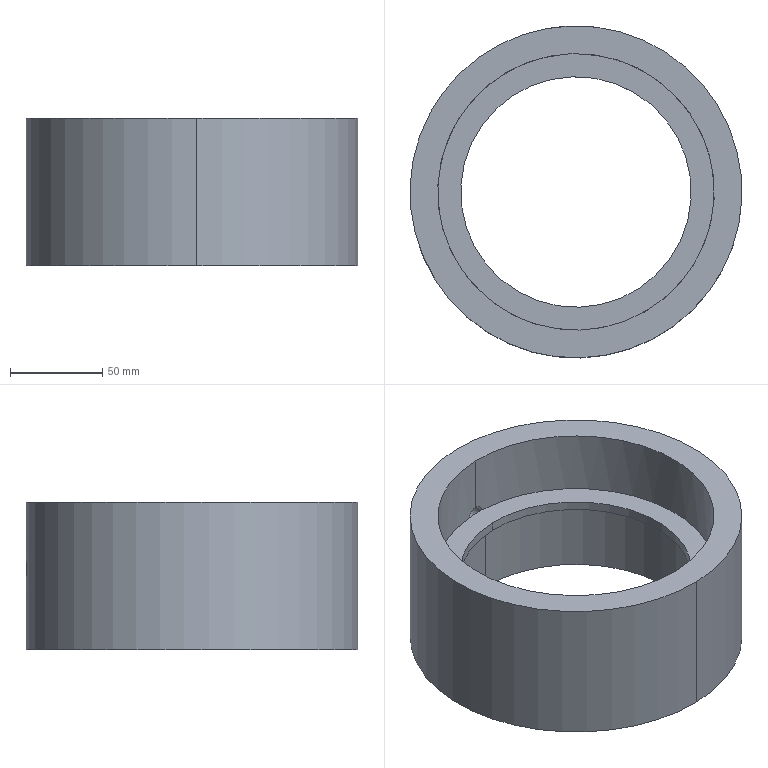Component | SolidWorks | BearingHousing-1 | 1 solid | 41 faces | volume 777654 mm3 | cylinder 25 | cone 12 | plane 4 | commonest cylinder face diameters 6.8 x12 150 x5 10.2 x2 135 x2 180 x2 125 x2 | material 45#